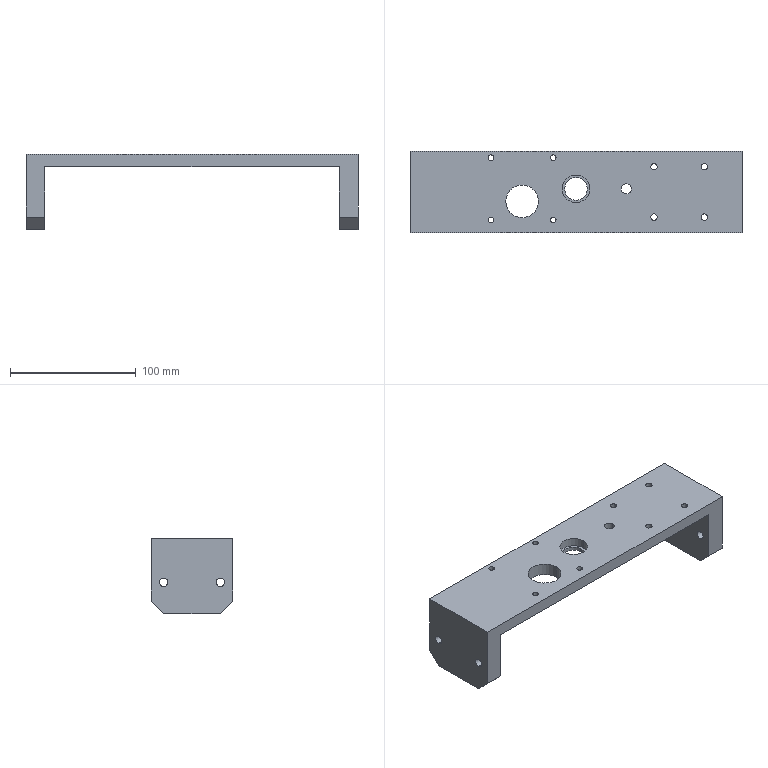CAM job | Mastercam | mm | 2 operations | part box 264 x 65 x 60
1. Contour (2D) | 10 - 10 平铣刀
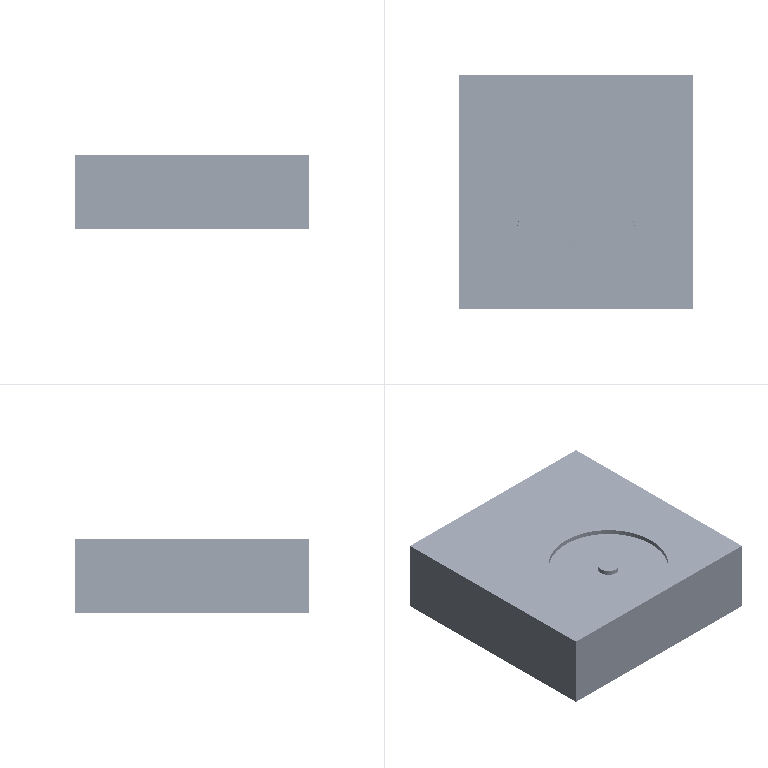2. Helix Bore | 3 - 3 平铣刀